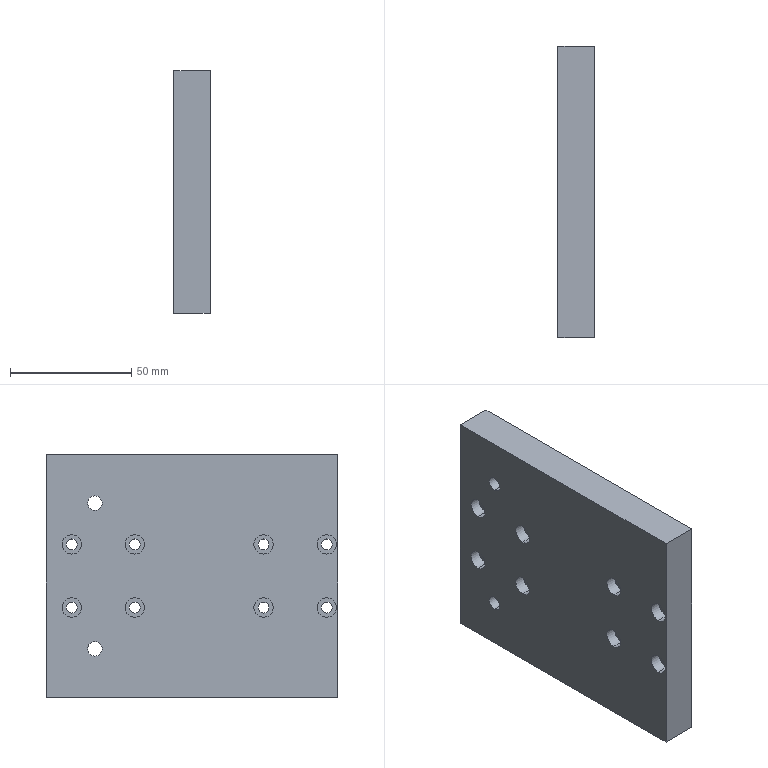Component | SolidWorks | SlideRailCarriage-1 | 1 solid | 50 faces | box 15.11 x 120 x 100.02 mm | volume 175979 mm3 | cylinder 36 | plane 14 | commonest cylinder face diameters 8 x16 4.5 x16 6 x4
build123d program:
from build123d import *

# Parameters (mm, degrees)
SKETCH1_W                                      = 120
SKETCH1_H                                      = 100
BOSS_EXTRUDE1_DEPTH                            = 15
M4_HEX_SOCKET_HEAD_CAP_SCREW_CBORE1_AT_2_COUNT = 2
M4_HEX_SOCKET_HEAD_CAP_SCREW_CBORE1_AT_2_PITCH = 26
M4_HEX_SOCKET_HEAD_CAP_SCREW_CBORE1_AT_3_COUNT = 2
M4_HEX_SOCKET_HEAD_CAP_SCREW_CBORE1_AT_3_PITCH = 26
M4_HEX_SOCKET_HEAD_CAP_SCREW_CBORE1_AT_4_COUNT = 2
M4_HEX_SOCKET_HEAD_CAP_SCREW_CBORE1_AT_4_PITCH = 36.77
M6_TAPPED_HOLE1_D                              = 6
M6_TAPPED_HOLE1_DEPTH                          = 15
M6_TAPPED_HOLE1_TIP                            = 1.803


with BuildPart() as part:
    # Sketch1 → Boss-Extrude1 (new body)
    with BuildSketch(Plane(origin=(0, 0, 0), x_dir=(1, 0, 0), z_dir=(0, 1, 0))):
        Rectangle(SKETCH1_W, SKETCH1_H)
    extrude(amount=BOSS_EXTRUDE1_DEPTH)

    # Sketch5 → M4 Hex Socket Head Cap Screw CBORE1 (revolve, cut)
    with BuildSketch(Plane(origin=(-49.571, 0, 13), x_dir=(0, 0, -1), z_dir=(1, 0, 0))):
        Polygon((0, 0), (0, 17.352), (2.25, 16), (2.25, 4.6), (4, 4.6), (4, 0), align=None)
    m4_hex_socket_head_cap_screw_cbore1 = revolve(axis=Axis((-49.571, -6.35, 13), (0, 1, 0)), mode=Mode.SUBTRACT)

    # M4 Hex Socket Head Cap Screw CBORE1 at 2: M4 Hex Socket Head Cap Screw CBORE1 ×2
    with Locations(*[(0, 0, -i * M4_HEX_SOCKET_HEAD_CAP_SCREW_CBORE1_AT_2_PITCH) for i in range(1, M4_HEX_SOCKET_HEAD_CAP_SCREW_CBORE1_AT_2_COUNT)]):
        add(m4_hex_socket_head_cap_screw_cbore1, mode=Mode.SUBTRACT)

    # M4 Hex Socket Head Cap Screw CBORE1 at 3: M4 Hex Socket Head Cap Screw CBORE1 ×2
    with Locations(*[(i * M4_HEX_SOCKET_HEAD_CAP_SCREW_CBORE1_AT_3_PITCH, 0, 0) for i in range(1, M4_HEX_SOCKET_HEAD_CAP_SCREW_CBORE1_AT_3_COUNT)]):
        add(m4_hex_socket_head_cap_screw_cbore1, mode=Mode.SUBTRACT)

    # M4 Hex Socket Head Cap Screw CBORE1 at 4: M4 Hex Socket Head Cap Screw CBORE1 ×2
    with Locations(*[Vector(0.7071, 0, -0.7071) * (i * M4_HEX_SOCKET_HEAD_CAP_SCREW_CBORE1_AT_4_PITCH) for i in range(1, M4_HEX_SOCKET_HEAD_CAP_SCREW_CBORE1_AT_4_COUNT)]):
        add(m4_hex_socket_head_cap_screw_cbore1, mode=Mode.SUBTRACT)

    # Mirror1: M4 Hex Socket Head Cap Screw CBORE1 across plane
    add(m4_hex_socket_head_cap_screw_cbore1.mirror(Plane(origin=(2.958, 0, 0), x_dir=(0, 0, 1), z_dir=(1, 0, 0))), mode=Mode.SUBTRACT)

    # Mirror1 copy 1 sketch → Mirror1 copy 1 (revolve, cut)
    with BuildSketch(Plane(origin=(55.487, 0, -13), x_dir=(0, 0, -1), z_dir=(-1, 0, 0))):
        Polygon((0, 0), (0, -17.352), (2.25, -16), (2.25, -4.6), (4, -4.6), (4, 0), align=None)
    revolve(axis=Axis((55.487, -6.35, -13), (0, -1, 0)), mode=Mode.SUBTRACT)

    # Mirror1 copy 2 sketch → Mirror1 copy 2 (revolve, cut)
    with BuildSketch(Plane(origin=(29.487, 0, 13), x_dir=(0, 0, -1), z_dir=(-1, 0, 0))):
        Polygon((0, 0), (0, -17.352), (2.25, -16), (2.25, -4.6), (4, -4.6), (4, 0), align=None)
    revolve(axis=Axis((29.487, -6.35, 13), (0, -1, 0)), mode=Mode.SUBTRACT)

    # Mirror1 copy 3 sketch → Mirror1 copy 3 (revolve, cut)
    with BuildSketch(Plane(origin=(29.487, 0, -13), x_dir=(0, 0, -1), z_dir=(-1, 0, 0))):
        Polygon((0, 0), (0, -17.352), (2.25, -16), (2.25, -4.6), (4, -4.6), (4, 0), align=None)
    revolve(axis=Axis((29.487, -6.35, -13), (0, -1, 0)), mode=Mode.SUBTRACT)

    # M6 Tapped Hole1
    with Locations(Plane(origin=(0, 0, 0), x_dir=(-1, 0, 0), z_dir=(0, -1, 0))):
        with Locations((40, 30), (40, -30)):
            Hole(M6_TAPPED_HOLE1_D / 2, depth=M6_TAPPED_HOLE1_DEPTH)
            with Locations((0, 0, -(M6_TAPPED_HOLE1_DEPTH + M6_TAPPED_HOLE1_TIP / 2))):  # 118° drill point
                Cone(0, M6_TAPPED_HOLE1_D / 2, M6_TAPPED_HOLE1_TIP, mode=Mode.SUBTRACT)


solid = part.part

# Placed as in the assembly
solid = solid.moved(Location((-80.542, 874.54, 1109.705), (0, 0.0619, -90)))